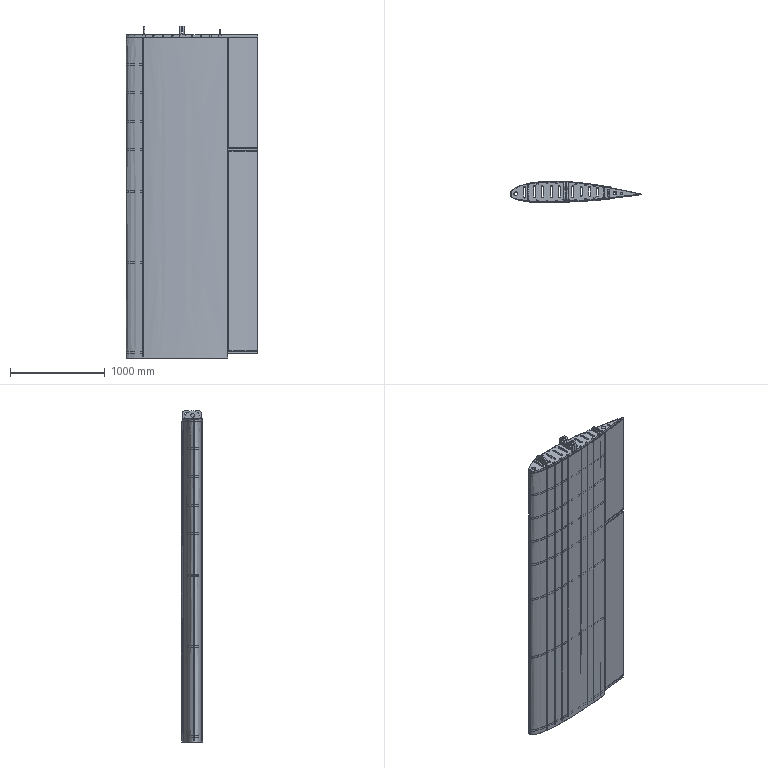Assembly | NX | mm | 53 component files | 53 solids | 2670 faces | box 1394.7 x 223.06 x 3513 mm | volume 23239674 mm3 | plane 1920 | cylinder 550 | other 104 | spline 96 | commonest cylinder face diameters 30 x167 20 x154 40 x70 13198.653 x32 8411.161 x32 13194.653 x32 8407.161 x32 122.237 x5
Bill of materials:
unnamed part 1 | 13 |  | Very thin planar C-shaped (three-sided open rectangular outline) sheet or surface, slightly rotated in its plane.
unnamed part 2 | 1 |  | Long, narrow, thin strip with a rounded end, a small hole near that end, and a long evenly spaced row of short transverse slots along its length.
unnamed part 3 | 8 |  | Flat plate, roughly rectangular, with slightly convex long edges, four parallel stadium-shaped through slots, and rectangular notches along both long edges that split the outline into four segments.
unnamed part 4 | 1 |  | Prism with a tapered teardrop profile (rounded wide end tapering to a point), extruded to a constant depth, with a larger hole near the rounded end and a small hole toward the tip.
unnamed part 5 | 8 |  | Flat tapered (trapezoidal) plate with slightly curved long edges, four parallel stadium slots that get shorter toward the narrow end, and rectangular notches along both long edges.
unnamed part 6 | 1 |  | Thin, gently curved rectangular sheet (a shallow single-curvature arc panel).
unnamed part 7 | 1 |  | Thin sheet bent into an open U- or parabola-shaped cross-section and extruded straight along its length.
unnamed part 8 | 1 |  | Prism with a tapered teardrop profile, extruded to a constant depth, with a large hole near the rounded end and a medium hole partway toward the tip.
unnamed part 9 | 5 |  | Thick plate or block with one straight edge and a large concave circular-arc cutout on the opposite side, with small offset steps on the straight side.
unnamed part 10 | 1 |  | Long, narrow, thin strip with a rounded end, a small hole near that end, and a long evenly spaced row of short transverse slots.
unnamed part 11 | 8 |  | Flat plate with an arched (ogive-like) outline and one straight edge, containing a large round hole, a long stadium slot parallel to the straight edge, and a small rectangular notch at the curved tip.
unnamed part 12 | 1 |  | Thin, gently curved rectangular sheet (a shallow arc panel).
unnamed part 13 | 3 |  | Flat plate of uniform thickness with a long tapered, roughly triangular outline. One end is wide and has small stepped notches at both corners; the other end narrows to a sharp point. Three through-cutouts sit along the centerline: an elongated slot near the wide end that runs across the width, then a larger round hole, then a smaller round hole.
unnamed part 14 | 1 |  | Long, narrow, thin strip with a single row of evenly spaced, rounded-end transverse slots (about 29) along most of its length. One end has two small rounded lobes or eyelets, each with a small hole, and the other end is plain and squared off.
Mates:
1. touch align | front_rib 8 face | mid_rib 8 face
2. touch align | front_rib 8 face | mid_rib 8 face
3. touch align | front_beam 1 face | mid_rib 8 face
4. touch align | front_beam 1 face | mid_rib 8 face
5. touch align | front_beam 1 face | mid_rib 8 face
6. touch align | front_rib 8 face | front_beam 1 face
7. touch align | mid_beam 1 face | mid_rib 8 face
8. touch align | mid_beam 1 face | mid_rib 8 face
9. touch align | mid_beam 1 face | mid_rib 8 face
10. touch align | mid_rear_rib 8 face | mid_beam 1 face
11. touch align | mid_rear_rib 8 face | mid_beam 1 face
12. touch align | mid_rear_rib 8 face | mid_beam 1 face
13. touch align | rear_beam 1 face | mid_rear_rib 8 face
14. touch align | rear_beam 1 face | mid_rear_rib 8 face
15. touch align | rear_beam 1 face | mid_rear_rib 8 face
16. touch align | rear_rib 3 face | rear_beam 1 face
17. touch align | rear_rib 3 face | rear_beam 1 face
18. touch align | rear_rib 3 face | rear_beam 1 face
19. bond | mid_rib 8 component | assembly component
20. bond | mid_rib 8 component | assembly component
21. bond | mid_rear_rib 8 component | assembly component
22. bond | front_rib 8 component | assembly component
23. bond | mid_rib 7 component | assembly component
24. bond | mid_rear_rib 7 component | assembly component
25. bond | front_rib 7 component | assembly component
26. linear | assembly datumaxis | assembly cartesiancoordinatesystem | assembly cartesiancoordinatesystem | assembly cartesiancoordinatesystem | assembly cartesiancoordinatesystem | assembly cartesiancoordinatesystem
27. linear | assembly datumaxis | assembly cartesiancoordinatesystem | assembly cartesiancoordinatesystem | assembly cartesiancoordinatesystem | assembly cartesiancoordinatesystem | assembly cartesiancoordinatesystem
28. linear | assembly datumaxis | assembly cartesiancoordinatesystem | assembly cartesiancoordinatesystem | assembly cartesiancoordinatesystem | assembly cartesiancoordinatesystem | assembly cartesiancoordinatesystem
29. bond | mid_rib 6 component | assembly component
30. bond | mid_rear_rib 6 component | assembly component
31. bond | front_rib 6 component | assembly component
32. bond | mid_rib 5 component | assembly component
33. bond | mid_rear_rib 5 component | assembly component
34. bond | front_rib 5 component | assembly component
35. bond | mid_rib 4 component | assembly component
36. bond | mid_rear_rib 4 component | assembly component
37. bond | front_rib 4 component | assembly component
38. bond | mid_rear_rib 4 component | assembly component
39. bond | front_rib 4 component | assembly component
40. bond | mid_rear_rib 4 component | assembly component
41. bond | mid_rib 4 component | assembly component
42. bond | front_rib 3 component | assembly component
43. bond | mid_rear_rib 3 component | assembly component
44. bond | mid_rib 3 component | assembly component
45. linear | assembly datumaxis | assembly cartesiancoordinatesystem | assembly cartesiancoordinatesystem
46. linear | assembly datumaxis | assembly cartesiancoordinatesystem | assembly cartesiancoordinatesystem
47. linear | assembly datumaxis | assembly cartesiancoordinatesystem | assembly cartesiancoordinatesystem
48. bond | mid_rib 3 component | assembly component
49. bond | front_rib 3 component | assembly component
50. bond | mid_rear_rib 3 component | assembly component
51. bond | mid_rib 3 component | assembly component
52. bond | front_rib 2 component | assembly component
53. bond | mid_rear_rib 2 component | assembly component
54. bond | mid_rib 2 component | assembly component
55. linear | assembly datumaxis | assembly cartesiancoordinatesystem | assembly cartesiancoordinatesystem
56. linear | assembly datumaxis | assembly cartesiancoordinatesystem | assembly cartesiancoordinatesystem
57. linear | assembly datumaxis | assembly cartesiancoordinatesystem | assembly cartesiancoordinatesystem
58. bond | mid_rear_rib 2 component | assembly component
59. bond | mid_rear_rib 2 component | assembly component
60. bond | front_rib 2 component | assembly component
61. bond | mid_rib 2 component | assembly component
62. bond | mid_rear_rib 1 component | assembly component
63. bond | front_rib 1 component | assembly component
64. bond | mid_rib 1 component | assembly component
65. linear | assembly datumaxis | assembly cartesiancoordinatesystem | assembly cartesiancoordinatesystem
66. linear | assembly datumaxis | assembly cartesiancoordinatesystem | assembly cartesiancoordinatesystem
67. linear | assembly datumaxis | assembly cartesiancoordinatesystem | assembly cartesiancoordinatesystem
68. bond | rear_rib 3 component | assembly component
69. bond | rear_rib 3 component | assembly component
70. bond | rear_rib 2 component | assembly component
71. linear | assembly datumaxis | assembly cartesiancoordinatesystem | assembly cartesiancoordinatesystem
72. bond | rear_rib 2 component | assembly component
73. bond | rear_rib 2 component | assembly component
74. bond | rear_rib 1 component | assembly component
75. linear | assembly datumaxis | assembly cartesiancoordinatesystem | assembly cartesiancoordinatesystem
76. touch align | flap_skin 1 face | rear_rib 3 face
77. distance | flap_skin 1 face | rear_rib 3 face
78. touch align | aileron_skin 1 face | rear_rib 2 face
79. distance | aileron_skin 1 face | rear_rib 2 face
80. touch align | aileron_rib 5 face | mid_rear_rib 7 face
81. touch align | aileron_rib 5 face | rear_beam 1 face
82. touch align | aileron_rib 5 face | rear_beam 1 face
83. bond | rear_beam 1 component | assembly component
84. bond | aileron_rib 5 component | assembly component
85. bond | aileron_rib 4 component | assembly component
86. linear | assembly datumaxis | assembly cartesiancoordinatesystem | assembly cartesiancoordinatesystem | assembly cartesiancoordinatesystem
87. bond | aileron_rib 3 component | assembly component
88. fix | assembly component
89. bond | aileron_rib 3 component | assembly component
90. bond | aileron_rib 2 component | assembly component
91. linear | assembly datumaxis | assembly cartesiancoordinatesystem | assembly cartesiancoordinatesystem
92. fix | assembly component
93. bond | aileron_rib 2 component | assembly component
94. bond | aileron_rib 1 component | assembly component
95. linear | assembly datumaxis | assembly cartesiancoordinatesystem | assembly cartesiancoordinatesystem
96. touch align | rib_strip 13 face | front_rib 8 face
97. touch align | rib_strip 13 face | front_rib 8 face
98. touch align | rib_strip 13 face | front_rib 8 face
99. touch align | rib_strip 12 face | mid_rib 8 face
100. touch align | rib_strip 12 face | mid_rib 8 face
101. touch align | rib_strip 7 face | mid_rear_rib 8 face
102. touch align | rib_strip 7 face | mid_rear_rib 8 face
103. touch align | rib_strip 8 face | mid_rear_rib 8 face
104. touch align | rib_strip 8 face | mid_rear_rib 8 face
105. touch align | rib_strip 9 face | mid_rear_rib 8 face
106. touch align | rib_strip 9 face | mid_rear_rib 8 face
107. touch align | rib_strip 10 face | mid_rib 8 face
108. touch align | rib_strip 10 face | mid_rib 8 face
109. touch align | rib_strip 11 face | mid_rib 8 face
110. fix | front_rib 8 component
111. touch align | rib_strip 11 face | mid_rib 8 face
112. touch align | rib_strip 2 face | mid_rear_rib 8 face
113. touch align | rib_strip 3 face | mid_rear_rib 8 face
114. touch align | rib_strip 6 face | mid_rear_rib 8 face
115. touch align | rib_strip 4 face | mid_rib 8 face
116. touch align | rib_strip 5 face | mid_rib 8 face
117. touch align | rib_strip 1 face | mid_rib 8 face
118. touch align | rib_strip 1 face | mid_rib 8 face
119. touch align | rib_strip 4 face | mid_rib 8 face
120. touch align | rib_strip 3 face | mid_rear_rib 8 face
121. touch align | rib_strip 6 face | mid_rear_rib 8 face
122. touch align | rib_strip 2 face | mid_rear_rib 8 face